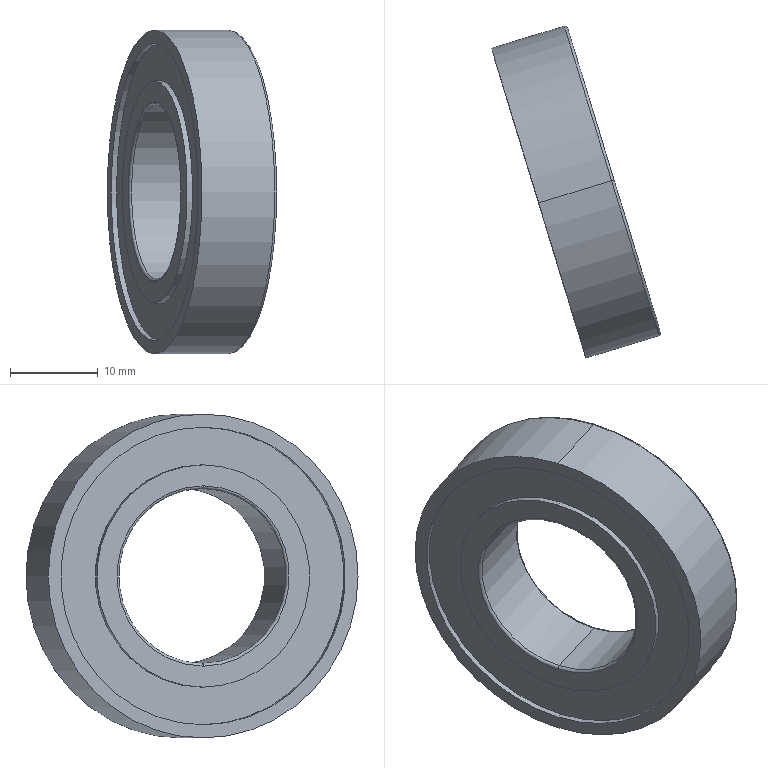Component | SolidWorks | v1ZHXTBGMWB6904ZZ_40SB1-1_v1ZHXTbearingB6904ZZSB1-1 | 1 solid | 24 faces | box 19.33 x 37.94 x 37 mm | volume 6323 mm3 | cylinder 12 | torus 6 | plane 6 | commonest cylinder face diameters 34 x4 25.4 x4 20 x2 37 x2
build123d program:
from build123d import *


with BuildPart() as part:
    # Sketch1 → Revolve1 (revolve)
    with BuildSketch(Plane.XY, mode=Mode.PRIVATE) as revolve1_sk:
        with BuildLine():
            Line((0, 18.5), (0, 17))
            Line((0, 17), (0.65, 17))
            Line((0.65, 17), (0.65, 12.7))
            Line((0.65, 12.7), (0, 12.7))
            Line((0, 12.7), (0, 10.3))
            ThreePointArc((0, 10.3), (0.08787, 10.088), (0.3, 10))
            Line((0.3, 10), (8.7, 10))
            ThreePointArc((8.7, 10), (8.912, 10.088), (9, 10.3))
            Line((9, 10.3), (9, 12.7))
            Line((9, 12.7), (8.35, 12.7))
            Line((8.35, 12.7), (8.35, 17))
            Line((8.35, 17), (9, 17))
            Line((9, 17), (9, 18.2))
            ThreePointArc((9, 18.2), (8.912, 18.412), (8.7, 18.5))
            Line((8.7, 18.5), (0, 18.5))
        make_face()
    revolve(revolve1_sk.sketch.rotate(Axis((9, 0, 0), (-1, 0, 0)), 270), axis=Axis((9, 0, 0), (-1, 0, 0)))


solid = part.part

# Placed as in the assembly
solid = solid.moved(Location((157.588, -238.137, 375.239), (15.285, 4.599, 16.35)))
STEP:
#1=CARTESIAN_POINT('',(6.543,-9.272,15.49));
#2=VERTEX_POINT('',#1);
#3=CARTESIAN_POINT('',(6.543,-9.272,14.057));
#4=VERTEX_POINT('',#3);
#5=CARTESIAN_POINT('',(6.543,-9.272,14.773));
#6=DIRECTION('',(-0.9565,-0.2918,-0.));
#7=DIRECTION('',(-0.,-0.,1.));
#8=AXIS2_PLACEMENT_3D('',#5,#6,#7);
#9=CIRCLE('',#8,0.7165);
#10=EDGE_CURVE('',#2,#4,#9,.T.);
#11=ORIENTED_EDGE('',*,*,#10,.T.);
#12=CARTESIAN_POINT('',(6.532,-9.276,14.045));
#13=VERTEX_POINT('',#12);
#14=CARTESIAN_POINT('',(6.532,-9.276,14.057));
#15=DIRECTION('',(-0.2918,0.9565,0.));
#16=DIRECTION('',(-0.9565,-0.2918,0.));
#17=AXIS2_PLACEMENT_3D('',#14,#15,#16);
#18=CIRCLE('',#17,0.01181);
#19=EDGE_CURVE('',#4,#13,#18,.T.);
#20=ORIENTED_EDGE('',*,*,#19,.T.);
#21=CARTESIAN_POINT('',(6.532,-9.276,15.502));
#22=VERTEX_POINT('',#21);
#23=CARTESIAN_POINT('',(6.532,-9.276,14.773));
#24=DIRECTION('',(-0.9565,-0.2918,-0.));
#25=DIRECTION('',(-0.,-0.,1.));
#26=AXIS2_PLACEMENT_3D('',#23,#24,#25);
#27=CIRCLE('',#26,0.7283);
#28=EDGE_CURVE('',#22,#13,#27,.T.);
#29=ORIENTED_EDGE('',*,*,#28,.F.);
#30=CARTESIAN_POINT('',(6.532,-9.276,15.49));
#31=DIRECTION('',(0.2918,-0.9565,-0.));
#32=DIRECTION('',(0.9565,0.2918,0.));
#33=AXIS2_PLACEMENT_3D('',#30,#31,#32);
#34=CIRCLE('',#33,0.01181);
#35=EDGE_CURVE('',#2,#22,#34,.T.);
#36=ORIENTED_EDGE('',*,*,#35,.F.);
#37=EDGE_LOOP('',(#11,#20,#29,#36));
#38=FACE_OUTER_BOUND('',#37,.T.);
#39=CARTESIAN_POINT('',(6.532,-9.276,14.773));
#40=DIRECTION('',(-0.9565,-0.2918,-0.));
#41=DIRECTION('',(-0.,-0.,1.));
#42=AXIS2_PLACEMENT_3D('',#39,#40,#41);
#43=TOROIDAL_SURFACE('',#42,0.7165,0.01181);
#44=ADVANCED_FACE('',(#38),#43,.T.);
#45=CARTESIAN_POINT('',(6.543,-9.272,14.104));
#46=VERTEX_POINT('',#45);
#47=CARTESIAN_POINT('',(6.543,-9.272,15.442));
#48=VERTEX_POINT('',#47);
#49=CARTESIAN_POINT('',(6.543,-9.272,14.773));
#50=DIRECTION('',(-0.9565,-0.2918,-0.));
#51=DIRECTION('',(-0.,-0.,1.));
#52=AXIS2_PLACEMENT_3D('',#49,#50,#51);
#53=CIRCLE('',#52,0.6693);
#54=EDGE_CURVE('',#46,#48,#53,.T.);
#55=ORIENTED_EDGE('',*,*,#54,.F.);
#56=CARTESIAN_POINT('',(6.519,-9.28,14.104));
#57=VERTEX_POINT('',#56);
#58=CARTESIAN_POINT('',(6.543,-9.272,14.104));
#59=DIRECTION('',(-0.9565,-0.2918,-0.));
#60=VECTOR('',#59,39.37);
#61=LINE('',#58,#60);
#62=EDGE_CURVE('',#46,#57,#61,.T.);
#63=ORIENTED_EDGE('',*,*,#62,.T.);
#64=CARTESIAN_POINT('',(6.519,-9.28,15.442));
#65=VERTEX_POINT('',#64);
#66=CARTESIAN_POINT('',(6.519,-9.28,14.773));
#67=DIRECTION('',(-0.9565,-0.2918,-0.));
#68=DIRECTION('',(-0.,-0.,1.));
#69=AXIS2_PLACEMENT_3D('',#66,#67,#68);
#70=CIRCLE('',#69,0.6693);
#71=EDGE_CURVE('',#57,#65,#70,.T.);
#72=ORIENTED_EDGE('',*,*,#71,.T.);
#73=CARTESIAN_POINT('',(6.543,-9.272,15.442));
#74=DIRECTION('',(-0.9565,-0.2918,-0.));
#75=VECTOR('',#74,39.37);
#76=LINE('',#73,#75);
#77=EDGE_CURVE('',#48,#65,#76,.T.);
#78=ORIENTED_EDGE('',*,*,#77,.F.);
#79=EDGE_LOOP('',(#55,#63,#72,#78));
#80=FACE_OUTER_BOUND('',#79,.T.);
#81=CARTESIAN_POINT('',(6.543,-9.272,14.773));
#82=DIRECTION('',(-0.9565,-0.2918,-0.));
#83=DIRECTION('',(-0.,-0.,1.));
#84=AXIS2_PLACEMENT_3D('',#81,#82,#83);
#85=CYLINDRICAL_SURFACE('',#84,0.6693);
#86=ADVANCED_FACE('',(#80),#85,.F.);
#87=CARTESIAN_POINT('',(6.543,-9.272,15.273));
#88=VERTEX_POINT('',#87);
#89=CARTESIAN_POINT('',(6.543,-9.272,14.273));
#90=VERTEX_POINT('',#89);
#91=CARTESIAN_POINT('',(6.543,-9.272,14.773));
#92=DIRECTION('',(-0.9565,-0.2918,-0.));
#93=DIRECTION('',(-0.,-0.,1.));
#94=AXIS2_PLACEMENT_3D('',#91,#92,#93);
#95=CIRCLE('',#94,0.5);
#96=EDGE_CURVE('',#88,#90,#95,.T.);
#97=ORIENTED_EDGE('',*,*,#96,.T.);
#98=CARTESIAN_POINT('',(6.519,-9.28,14.273));
#99=VERTEX_POINT('',#98);
#100=CARTESIAN_POINT('',(6.543,-9.272,14.273));
#101=DIRECTION('',(-0.9565,-0.2918,-0.));
#102=VECTOR('',#101,39.37);
#103=LINE('',#100,#102);
#104=EDGE_CURVE('',#90,#99,#103,.T.);
#105=ORIENTED_EDGE('',*,*,#104,.T.);
#106=CARTESIAN_POINT('',(6.519,-9.28,15.273));
#107=VERTEX_POINT('',#106);
#108=CARTESIAN_POINT('',(6.519,-9.28,14.773));
#109=DIRECTION('',(-0.9565,-0.2918,-0.));
#110=DIRECTION('',(-0.,-0.,1.));
#111=AXIS2_PLACEMENT_3D('',#108,#109,#110);
#112=CIRCLE('',#111,0.5);
#113=EDGE_CURVE('',#107,#99,#112,.T.);
#114=ORIENTED_EDGE('',*,*,#113,.F.);
#115=CARTESIAN_POINT('',(6.543,-9.272,15.273));
#116=DIRECTION('',(-0.9565,-0.2918,-0.));
#117=VECTOR('',#116,39.37);
#118=LINE('',#115,#117);
#119=EDGE_CURVE('',#88,#107,#118,.T.);
#120=ORIENTED_EDGE('',*,*,#119,.F.);
#121=EDGE_LOOP('',(#97,#105,#114,#120));
#122=FACE_OUTER_BOUND('',#121,.T.);
#123=CARTESIAN_POINT('',(6.543,-9.272,14.773));
#124=DIRECTION('',(-0.9565,-0.2918,-0.));
#125=DIRECTION('',(-0.,-0.,1.));
#126=AXIS2_PLACEMENT_3D('',#123,#124,#125);
#127=CYLINDRICAL_SURFACE('',#126,0.5);
#128=ADVANCED_FACE('',(#122),#127,.T.);
#129=CARTESIAN_POINT('',(6.532,-9.276,15.167));
#130=VERTEX_POINT('',#129);
#131=CARTESIAN_POINT('',(6.532,-9.276,14.379));
#132=VERTEX_POINT('',#131);
#133=CARTESIAN_POINT('',(6.532,-9.276,14.773));
#134=DIRECTION('',(-0.9565,-0.2918,-0.));
#135=DIRECTION('',(0.,-0.,1.));
#136=AXIS2_PLACEMENT_3D('',#133,#134,#135);
#137=CIRCLE('',#136,0.3937);
#138=EDGE_CURVE('',#130,#132,#137,.T.);
#139=ORIENTED_EDGE('',*,*,#138,.T.);
#140=CARTESIAN_POINT('',(6.543,-9.272,14.368));
#141=VERTEX_POINT('',#140);
#142=CARTESIAN_POINT('',(6.532,-9.276,14.368));
#143=DIRECTION('',(-0.2918,0.9565,0.));
#144=DIRECTION('',(-0.9565,-0.2918,0.));
#145=AXIS2_PLACEMENT_3D('',#142,#143,#144);
#146=CIRCLE('',#145,0.01181);
#147=EDGE_CURVE('',#132,#141,#146,.T.);
#148=ORIENTED_EDGE('',*,*,#147,.T.);
#149=CARTESIAN_POINT('',(6.543,-9.272,15.179));
#150=VERTEX_POINT('',#149);
#151=CARTESIAN_POINT('',(6.543,-9.272,14.773));
#152=DIRECTION('',(-0.9565,-0.2918,-0.));
#153=DIRECTION('',(-0.,-0.,1.));
#154=AXIS2_PLACEMENT_3D('',#151,#152,#153);
#155=CIRCLE('',#154,0.4055);
#156=EDGE_CURVE('',#150,#141,#155,.T.);
#157=ORIENTED_EDGE('',*,*,#156,.F.);
#158=CARTESIAN_POINT('',(6.532,-9.276,15.179));
#159=DIRECTION('',(0.2918,-0.9565,-0.));
#160=DIRECTION('',(0.9565,0.2918,0.));
#161=AXIS2_PLACEMENT_3D('',#158,#159,#160);
#162=CIRCLE('',#161,0.01181);
#163=EDGE_CURVE('',#130,#150,#162,.T.);
#164=ORIENTED_EDGE('',*,*,#163,.F.);
#165=EDGE_LOOP('',(#139,#148,#157,#164));
#166=FACE_OUTER_BOUND('',#165,.T.);
#167=CARTESIAN_POINT('',(6.532,-9.276,14.773));
#168=DIRECTION('',(-0.9565,-0.2918,-0.));
#169=DIRECTION('',(-0.,-0.,1.));
#170=AXIS2_PLACEMENT_3D('',#167,#168,#169);
#171=TOROIDAL_SURFACE('',#170,0.4055,0.01181);
#172=ADVANCED_FACE('',(#166),#171,.T.);
#173=CARTESIAN_POINT('',(6.532,-9.276,14.773));
#174=DIRECTION('',(-0.9565,-0.2918,-0.));
#175=DIRECTION('',(0.,-0.,1.));
#176=AXIS2_PLACEMENT_3D('',#173,#174,#175);
#177=CIRCLE('',#176,0.3937);
#178=EDGE_CURVE('',#132,#130,#177,.T.);
#179=ORIENTED_EDGE('',*,*,#178,.F.);
#180=CARTESIAN_POINT('',(6.216,-9.372,14.379));
#181=VERTEX_POINT('',#180);
#182=CARTESIAN_POINT('',(6.543,-9.272,14.379));
#183=DIRECTION('',(-0.9565,-0.2918,-0.));
#184=VECTOR('',#183,39.37);
#185=LINE('',#182,#184);
#186=EDGE_CURVE('',#132,#181,#185,.T.);
#187=ORIENTED_EDGE('',*,*,#186,.T.);
#188=CARTESIAN_POINT('',(6.216,-9.372,15.167));
#189=VERTEX_POINT('',#188);
#190=CARTESIAN_POINT('',(6.216,-9.372,14.773));
#191=DIRECTION('',(-0.9565,-0.2918,-0.));
#192=DIRECTION('',(0.,-0.,1.));
#193=AXIS2_PLACEMENT_3D('',#190,#191,#192);
#194=CIRCLE('',#193,0.3937);
#195=EDGE_CURVE('',#181,#189,#194,.T.);
#196=ORIENTED_EDGE('',*,*,#195,.T.);
#197=CARTESIAN_POINT('',(6.543,-9.272,15.167));
#198=DIRECTION('',(-0.9565,-0.2918,-0.));
#199=VECTOR('',#198,39.37);
#200=LINE('',#197,#199);
#201=EDGE_CURVE('',#130,#189,#200,.T.);
#202=ORIENTED_EDGE('',*,*,#201,.F.);
#203=EDGE_LOOP('',(#179,#187,#196,#202));
#204=FACE_OUTER_BOUND('',#203,.T.);
#205=CARTESIAN_POINT('',(6.543,-9.272,14.773));
#206=DIRECTION('',(-0.9565,-0.2918,-0.));
#207=DIRECTION('',(0.,-0.,1.));
#208=AXIS2_PLACEMENT_3D('',#205,#206,#207);
#209=CYLINDRICAL_SURFACE('',#208,0.3937);
#210=ADVANCED_FACE('',(#204),#209,.F.);
#211=CARTESIAN_POINT('',(6.204,-9.375,15.179));
#212=VERTEX_POINT('',#211);
#213=CARTESIAN_POINT('',(6.204,-9.375,14.368));
#214=VERTEX_POINT('',#213);
#215=CARTESIAN_POINT('',(6.204,-9.375,14.773));
#216=DIRECTION('',(-0.9565,-0.2918,-0.));
#217=DIRECTION('',(-0.,-0.,1.));
#218=AXIS2_PLACEMENT_3D('',#215,#216,#217);
#219=CIRCLE('',#218,0.4055);
#220=EDGE_CURVE('',#212,#214,#219,.T.);
#221=ORIENTED_EDGE('',*,*,#220,.T.);
#222=CARTESIAN_POINT('',(6.216,-9.372,14.368));
#223=DIRECTION('',(-0.2918,0.9565,0.));
#224=DIRECTION('',(-0.9565,-0.2918,0.));
#225=AXIS2_PLACEMENT_3D('',#222,#223,#224);
#226=CIRCLE('',#225,0.01181);
#227=EDGE_CURVE('',#214,#181,#226,.T.);
#228=ORIENTED_EDGE('',*,*,#227,.T.);
#229=CARTESIAN_POINT('',(6.216,-9.372,14.773));
#230=DIRECTION('',(-0.9565,-0.2918,-0.));
#231=DIRECTION('',(0.,-0.,1.));
#232=AXIS2_PLACEMENT_3D('',#229,#230,#231);
#233=CIRCLE('',#232,0.3937);
#234=EDGE_CURVE('',#189,#181,#233,.T.);
#235=ORIENTED_EDGE('',*,*,#234,.F.);
#236=CARTESIAN_POINT('',(6.216,-9.372,15.179));
#237=DIRECTION('',(0.2918,-0.9565,-0.));
#238=DIRECTION('',(0.9565,0.2918,0.));
#239=AXIS2_PLACEMENT_3D('',#236,#237,#238);
#240=CIRCLE('',#239,0.01181);
#241=EDGE_CURVE('',#212,#189,#240,.T.);
#242=ORIENTED_EDGE('',*,*,#241,.F.);
#243=EDGE_LOOP('',(#221,#228,#235,#242));
#244=FACE_OUTER_BOUND('',#243,.T.);
#245=CARTESIAN_POINT('',(6.216,-9.372,14.773));
#246=DIRECTION('',(-0.9565,-0.2918,-0.));
#247=DIRECTION('',(-0.,-0.,1.));
#248=AXIS2_PLACEMENT_3D('',#245,#246,#247);
#249=TOROIDAL_SURFACE('',#248,0.4055,0.01181);
#250=ADVANCED_FACE('',(#244),#249,.T.);
#251=CARTESIAN_POINT('',(6.229,-9.368,15.273));
#252=VERTEX_POINT('',#251);
#253=CARTESIAN_POINT('',(6.229,-9.368,14.273));
#254=VERTEX_POINT('',#253);
#255=CARTESIAN_POINT('',(6.229,-9.368,14.773));
#256=DIRECTION('',(-0.9565,-0.2918,-0.));
#257=DIRECTION('',(-0.,-0.,1.));
#258=AXIS2_PLACEMENT_3D('',#255,#256,#257);
#259=CIRCLE('',#258,0.5);
#260=EDGE_CURVE('',#252,#254,#259,.T.);
#261=ORIENTED_EDGE('',*,*,#260,.T.);
#262=CARTESIAN_POINT('',(6.204,-9.375,14.273));
#263=VERTEX_POINT('',#262);
#264=CARTESIAN_POINT('',(6.543,-9.272,14.273));
#265=DIRECTION('',(-0.9565,-0.2918,-0.));
#266=VECTOR('',#265,39.37);
#267=LINE('',#264,#266);
#268=EDGE_CURVE('',#254,#263,#267,.T.);
#269=ORIENTED_EDGE('',*,*,#268,.T.);
#270=CARTESIAN_POINT('',(6.204,-9.375,15.273));
#271=VERTEX_POINT('',#270);
#272=CARTESIAN_POINT('',(6.204,-9.375,14.773));
#273=DIRECTION('',(-0.9565,-0.2918,-0.));
#274=DIRECTION('',(-0.,-0.,1.));
#275=AXIS2_PLACEMENT_3D('',#272,#273,#274);
#276=CIRCLE('',#275,0.5);
#277=EDGE_CURVE('',#271,#263,#276,.T.);
#278=ORIENTED_EDGE('',*,*,#277,.F.);
#279=CARTESIAN_POINT('',(6.543,-9.272,15.273));
#280=DIRECTION('',(-0.9565,-0.2918,-0.));
#281=VECTOR('',#280,39.37);
#282=LINE('',#279,#281);
#283=EDGE_CURVE('',#252,#271,#282,.T.);
#284=ORIENTED_EDGE('',*,*,#283,.F.);
#285=EDGE_LOOP('',(#261,#269,#278,#284));
#286=FACE_OUTER_BOUND('',#285,.T.);
#287=CARTESIAN_POINT('',(6.543,-9.272,14.773));
#288=DIRECTION('',(-0.9565,-0.2918,-0.));
#289=DIRECTION('',(-0.,-0.,1.));
#290=AXIS2_PLACEMENT_3D('',#287,#288,#289);
#291=CYLINDRICAL_SURFACE('',#290,0.5);
#292=ADVANCED_FACE('',(#286),#291,.T.);
#293=CARTESIAN_POINT('',(6.229,-9.368,14.104));
#294=VERTEX_POINT('',#293);
#295=CARTESIAN_POINT('',(6.229,-9.368,15.442));
#296=VERTEX_POINT('',#295);
#297=CARTESIAN_POINT('',(6.229,-9.368,14.773));
#298=DIRECTION('',(-0.9565,-0.2918,-0.));
#299=DIRECTION('',(-0.,-0.,1.));
#300=AXIS2_PLACEMENT_3D('',#297,#298,#299);
#301=CIRCLE('',#300,0.6693);
#302=EDGE_CURVE('',#294,#296,#301,.T.);
#303=ORIENTED_EDGE('',*,*,#302,.F.);
#304=CARTESIAN_POINT('',(6.204,-9.375,14.104));
#305=VERTEX_POINT('',#304);
#306=CARTESIAN_POINT('',(6.543,-9.272,14.104));
#307=DIRECTION('',(-0.9565,-0.2918,-0.));
#308=VECTOR('',#307,39.37);
#309=LINE('',#306,#308);
#310=EDGE_CURVE('',#294,#305,#309,.T.);
#311=ORIENTED_EDGE('',*,*,#310,.T.);
#312=CARTESIAN_POINT('',(6.204,-9.375,15.442));
#313=VERTEX_POINT('',#312);
#314=CARTESIAN_POINT('',(6.204,-9.375,14.773));
#315=DIRECTION('',(-0.9565,-0.2918,-0.));
#316=DIRECTION('',(-0.,-0.,1.));
#317=AXIS2_PLACEMENT_3D('',#314,#315,#316);
#318=CIRCLE('',#317,0.6693);
#319=EDGE_CURVE('',#305,#313,#318,.T.);
#320=ORIENTED_EDGE('',*,*,#319,.T.);
#321=CARTESIAN_POINT('',(6.543,-9.272,15.442));
#322=DIRECTION('',(-0.9565,-0.2918,-0.));
#323=VECTOR('',#322,39.37);
#324=LINE('',#321,#323);
#325=EDGE_CURVE('',#296,#313,#324,.T.);
#326=ORIENTED_EDGE('',*,*,#325,.F.);
#327=EDGE_LOOP('',(#303,#311,#320,#326));
#328=FACE_OUTER_BOUND('',#327,.T.);
#329=CARTESIAN_POINT('',(6.543,-9.272,14.773));
#330=DIRECTION('',(-0.9565,-0.2918,-0.));
#331=DIRECTION('',(-0.,-0.,1.));
#332=AXIS2_PLACEMENT_3D('',#329,#330,#331);
#333=CYLINDRICAL_SURFACE('',#332,0.6693);
#334=ADVANCED_FACE('',(#328),#333,.F.);
#335=ORIENTED_EDGE('',*,*,#28,.T.);
#336=CARTESIAN_POINT('',(6.204,-9.375,14.045));
#337=VERTEX_POINT('',#336);
#338=CARTESIAN_POINT('',(6.543,-9.272,14.045));
#339=DIRECTION('',(-0.9565,-0.2918,-0.));
#340=VECTOR('',#339,39.37);
#341=LINE('',#338,#340);
#342=EDGE_CURVE('',#13,#337,#341,.T.);
#343=ORIENTED_EDGE('',*,*,#342,.T.);
#344=CARTESIAN_POINT('',(6.204,-9.375,15.502));
#345=VERTEX_POINT('',#344);
#346=CARTESIAN_POINT('',(6.204,-9.375,14.773));
#347=DIRECTION('',(-0.9565,-0.2918,-0.));
#348=DIRECTION('',(-0.,-0.,1.));
#349=AXIS2_PLACEMENT_3D('',#346,#347,#348);
#350=CIRCLE('',#349,0.7283);
#351=EDGE_CURVE('',#345,#337,#350,.T.);
#352=ORIENTED_EDGE('',*,*,#351,.F.);
#353=CARTESIAN_POINT('',(6.543,-9.272,15.502));
#354=DIRECTION('',(-0.9565,-0.2918,-0.));
#355=VECTOR('',#354,39.37);
#356=LINE('',#353,#355);
#357=EDGE_CURVE('',#22,#345,#356,.T.);
#358=ORIENTED_EDGE('',*,*,#357,.F.);
#359=EDGE_LOOP('',(#335,#343,#352,#358));
#360=FACE_OUTER_BOUND('',#359,.T.);
#361=CARTESIAN_POINT('',(6.543,-9.272,14.773));
#362=DIRECTION('',(-0.9565,-0.2918,-0.));
#363=DIRECTION('',(-0.,-0.,1.));
#364=AXIS2_PLACEMENT_3D('',#361,#362,#363);
#365=CYLINDRICAL_SURFACE('',#364,0.7283);
#366=ADVANCED_FACE('',(#360),#365,.T.);
#367=ORIENTED_EDGE('',*,*,#342,.F.);
#368=CARTESIAN_POINT('',(6.532,-9.276,14.773));
#369=DIRECTION('',(-0.9565,-0.2918,-0.));
#370=DIRECTION('',(-0.,-0.,1.));
#371=AXIS2_PLACEMENT_3D('',#368,#369,#370);
#372=CIRCLE('',#371,0.7283);
#373=EDGE_CURVE('',#13,#22,#372,.T.);
#374=ORIENTED_EDGE('',*,*,#373,.T.);
#375=ORIENTED_EDGE('',*,*,#357,.T.);
#376=CARTESIAN_POINT('',(6.204,-9.375,14.773));
#377=DIRECTION('',(-0.9565,-0.2918,-0.));
#378=DIRECTION('',(-0.,-0.,1.));
#379=AXIS2_PLACEMENT_3D('',#376,#377,#378);
#380=CIRCLE('',#379,0.7283);
#381=EDGE_CURVE('',#337,#345,#380,.T.);
#382=ORIENTED_EDGE('',*,*,#381,.F.);
#383=EDGE_LOOP('',(#367,#374,#375,#382));
#384=FACE_OUTER_BOUND('',#383,.T.);
#385=CARTESIAN_POINT('',(6.543,-9.272,14.773));
#386=DIRECTION('',(-0.9565,-0.2918,-0.));
#387=DIRECTION('',(-0.,-0.,1.));
#388=AXIS2_PLACEMENT_3D('',#385,#386,#387);
#389=CYLINDRICAL_SURFACE('',#388,0.7283);
#390=ADVANCED_FACE('',(#384),#389,.T.);
#391=CARTESIAN_POINT('',(6.204,-9.375,14.773));
#392=DIRECTION('',(-0.9565,-0.2918,-0.));
#393=DIRECTION('',(-0.,-0.,1.));
#394=AXIS2_PLACEMENT_3D('',#391,#392,#393);
#395=CIRCLE('',#394,0.6693);
#396=EDGE_CURVE('',#313,#305,#395,.T.);
#397=ORIENTED_EDGE('',*,*,#396,.F.);
#398=ORIENTED_EDGE('',*,*,#319,.F.);
#399=EDGE_LOOP('',(#397,#398));
#400=FACE_BOUND('',#399,.T.);
#401=ORIENTED_EDGE('',*,*,#351,.T.);
#402=ORIENTED_EDGE('',*,*,#381,.T.);
#403=EDGE_LOOP('',(#401,#402));
#404=FACE_OUTER_BOUND('',#403,.T.);
#405=CARTESIAN_POINT('',(5.992,-8.679,14.773));
#406=DIRECTION('',(0.9565,0.2918,0.));
#407=DIRECTION('',(0.,0.,-1.));
#408=AXIS2_PLACEMENT_3D('',#405,#406,#407);
#409=PLANE('',#408);
#410=ADVANCED_FACE('',(#400,#404),#409,.F.);
#411=ORIENTED_EDGE('',*,*,#310,.F.);
#412=CARTESIAN_POINT('',(6.229,-9.368,14.773));
#413=DIRECTION('',(-0.9565,-0.2918,-0.));
#414=DIRECTION('',(-0.,-0.,1.));
#415=AXIS2_PLACEMENT_3D('',#412,#413,#414);
#416=CIRCLE('',#415,0.6693);
#417=EDGE_CURVE('',#296,#294,#416,.T.);
#418=ORIENTED_EDGE('',*,*,#417,.F.);
#419=ORIENTED_EDGE('',*,*,#325,.T.);
#420=ORIENTED_EDGE('',*,*,#396,.T.);
#421=EDGE_LOOP('',(#411,#418,#419,#420));
#422=FACE_OUTER_BOUND('',#421,.T.);
#423=CARTESIAN_POINT('',(6.543,-9.272,14.773));
#424=DIRECTION('',(-0.9565,-0.2918,-0.));
#425=DIRECTION('',(-0.,-0.,1.));
#426=AXIS2_PLACEMENT_3D('',#423,#424,#425);
#427=CYLINDRICAL_SURFACE('',#426,0.6693);
#428=ADVANCED_FACE('',(#422),#427,.F.);
#429=ORIENTED_EDGE('',*,*,#260,.F.);
#430=CARTESIAN_POINT('',(6.229,-9.368,14.773));
#431=DIRECTION('',(-0.9565,-0.2918,-0.));
#432=DIRECTION('',(-0.,-0.,1.));
#433=AXIS2_PLACEMENT_3D('',#430,#431,#432);
#434=CIRCLE('',#433,0.5);
#435=EDGE_CURVE('',#254,#252,#434,.T.);
#436=ORIENTED_EDGE('',*,*,#435,.F.);
#437=EDGE_LOOP('',(#429,#436));
#438=FACE_BOUND('',#437,.T.);
#439=ORIENTED_EDGE('',*,*,#417,.T.);
#440=ORIENTED_EDGE('',*,*,#302,.T.);
#441=EDGE_LOOP('',(#439,#440));
#442=FACE_OUTER_BOUND('',#441,.T.);
#443=CARTESIAN_POINT('',(6.033,-8.728,14.773));
#444=DIRECTION('',(0.9565,0.2918,0.));
#445=DIRECTION('',(0.,0.,-1.));
#446=AXIS2_PLACEMENT_3D('',#443,#444,#445);
#447=PLANE('',#446);
#448=ADVANCED_FACE('',(#438,#442),#447,.F.);
#449=ORIENTED_EDGE('',*,*,#268,.F.);
#450=ORIENTED_EDGE('',*,*,#435,.T.);
#451=ORIENTED_EDGE('',*,*,#283,.T.);
#452=CARTESIAN_POINT('',(6.204,-9.375,14.773));
#453=DIRECTION('',(-0.9565,-0.2918,-0.));
#454=DIRECTION('',(-0.,-0.,1.));
#455=AXIS2_PLACEMENT_3D('',#452,#453,#454);
#456=CIRCLE('',#455,0.5);
#457=EDGE_CURVE('',#263,#271,#456,.T.);
#458=ORIENTED_EDGE('',*,*,#457,.F.);
#459=EDGE_LOOP('',(#449,#450,#451,#458));
#460=FACE_OUTER_BOUND('',#459,.T.);
#461=CARTESIAN_POINT('',(6.543,-9.272,14.773));
#462=DIRECTION('',(-0.9565,-0.2918,-0.));
#463=DIRECTION('',(-0.,-0.,1.));
#464=AXIS2_PLACEMENT_3D('',#461,#462,#463);
#465=CYLINDRICAL_SURFACE('',#464,0.5);
#466=ADVANCED_FACE('',(#460),#465,.T.);
#467=ORIENTED_EDGE('',*,*,#220,.F.);
#468=CARTESIAN_POINT('',(6.204,-9.375,14.773));
#469=DIRECTION('',(-0.9565,-0.2918,-0.));
#470=DIRECTION('',(-0.,-0.,1.));
#471=AXIS2_PLACEMENT_3D('',#468,#469,#470);
#472=CIRCLE('',#471,0.4055);
#473=EDGE_CURVE('',#214,#212,#472,.T.);
#474=ORIENTED_EDGE('',*,*,#473,.F.);
#475=EDGE_LOOP('',(#467,#474));
#476=FACE_BOUND('',#475,.T.);
#477=ORIENTED_EDGE('',*,*,#277,.T.);
#478=ORIENTED_EDGE('',*,*,#457,.T.);
#479=EDGE_LOOP('',(#477,#478));
#480=FACE_OUTER_BOUND('',#479,.T.);
#481=CARTESIAN_POINT('',(6.058,-8.897,14.773));
#482=DIRECTION('',(0.9565,0.2918,0.));
#483=DIRECTION('',(0.,0.,-1.));
#484=AXIS2_PLACEMENT_3D('',#481,#482,#483);
#485=PLANE('',#484);
#486=ADVANCED_FACE('',(#476,#480),#485,.F.);
#487=ORIENTED_EDGE('',*,*,#227,.F.);
#488=ORIENTED_EDGE('',*,*,#473,.T.);
#489=ORIENTED_EDGE('',*,*,#241,.T.);
#490=ORIENTED_EDGE('',*,*,#195,.F.);
#491=EDGE_LOOP('',(#487,#488,#489,#490));
#492=FACE_OUTER_BOUND('',#491,.T.);
#493=CARTESIAN_POINT('',(6.216,-9.372,14.773));
#494=DIRECTION('',(-0.9565,-0.2918,-0.));
#495=DIRECTION('',(-0.,-0.,1.));
#496=AXIS2_PLACEMENT_3D('',#493,#494,#495);
#497=TOROIDAL_SURFACE('',#496,0.4055,0.01181);
#498=ADVANCED_FACE('',(#492),#497,.T.);
#499=ORIENTED_EDGE('',*,*,#186,.F.);
#500=ORIENTED_EDGE('',*,*,#138,.F.);
#501=ORIENTED_EDGE('',*,*,#201,.T.);
#502=ORIENTED_EDGE('',*,*,#234,.T.);
#503=EDGE_LOOP('',(#499,#500,#501,#502));
#504=FACE_OUTER_BOUND('',#503,.T.);
#505=CARTESIAN_POINT('',(6.543,-9.272,14.773));
#506=DIRECTION('',(-0.9565,-0.2918,-0.));
#507=DIRECTION('',(0.,-0.,1.));
#508=AXIS2_PLACEMENT_3D('',#505,#506,#507);
#509=CYLINDRICAL_SURFACE('',#508,0.3937);
#510=ADVANCED_FACE('',(#504),#509,.F.);
#511=ORIENTED_EDGE('',*,*,#147,.F.);
#512=ORIENTED_EDGE('',*,*,#178,.T.);
#513=ORIENTED_EDGE('',*,*,#163,.T.);
#514=CARTESIAN_POINT('',(6.543,-9.272,14.773));
#515=DIRECTION('',(-0.9565,-0.2918,-0.));
#516=DIRECTION('',(-0.,-0.,1.));
#517=AXIS2_PLACEMENT_3D('',#514,#515,#516);
#518=CIRCLE('',#517,0.4055);
#519=EDGE_CURVE('',#141,#150,#518,.T.);
#520=ORIENTED_EDGE('',*,*,#519,.F.);
#521=EDGE_LOOP('',(#511,#512,#513,#520));
#522=FACE_OUTER_BOUND('',#521,.T.);
#523=CARTESIAN_POINT('',(6.532,-9.276,14.773));
#524=DIRECTION('',(-0.9565,-0.2918,-0.));
#525=DIRECTION('',(-0.,-0.,1.));
#526=AXIS2_PLACEMENT_3D('',#523,#524,#525);
#527=TOROIDAL_SURFACE('',#526,0.4055,0.01181);
#528=ADVANCED_FACE('',(#522),#527,.T.);
#529=ORIENTED_EDGE('',*,*,#96,.F.);
#530=CARTESIAN_POINT('',(6.543,-9.272,14.773));
#531=DIRECTION('',(-0.9565,-0.2918,-0.));
#532=DIRECTION('',(-0.,-0.,1.));
#533=AXIS2_PLACEMENT_3D('',#530,#531,#532);
#534=CIRCLE('',#533,0.5);
#535=EDGE_CURVE('',#90,#88,#534,.T.);
#536=ORIENTED_EDGE('',*,*,#535,.F.);
#537=EDGE_LOOP('',(#529,#536));
#538=FACE_OUTER_BOUND('',#537,.T.);
#539=ORIENTED_EDGE('',*,*,#156,.T.);
#540=ORIENTED_EDGE('',*,*,#519,.T.);
#541=EDGE_LOOP('',(#539,#540));
#542=FACE_BOUND('',#541,.T.);
#543=CARTESIAN_POINT('',(6.425,-8.884,14.773));
#544=DIRECTION('',(-0.9565,-0.2918,-0.));
#545=DIRECTION('',(-0.,-0.,1.));
#546=AXIS2_PLACEMENT_3D('',#543,#544,#545);
#547=PLANE('',#546);
#548=ADVANCED_FACE('',(#538,#542),#547,.F.);
#549=ORIENTED_EDGE('',*,*,#104,.F.);
#550=ORIENTED_EDGE('',*,*,#535,.T.);
#551=ORIENTED_EDGE('',*,*,#119,.T.);
#552=CARTESIAN_POINT('',(6.519,-9.28,14.773));
#553=DIRECTION('',(-0.9565,-0.2918,-0.));
#554=DIRECTION('',(-0.,-0.,1.));
#555=AXIS2_PLACEMENT_3D('',#552,#553,#554);
#556=CIRCLE('',#555,0.5);
#557=EDGE_CURVE('',#99,#107,#556,.T.);
#558=ORIENTED_EDGE('',*,*,#557,.F.);
#559=EDGE_LOOP('',(#549,#550,#551,#558));
#560=FACE_OUTER_BOUND('',#559,.T.);
#561=CARTESIAN_POINT('',(6.543,-9.272,14.773));
#562=DIRECTION('',(-0.9565,-0.2918,-0.));
#563=DIRECTION('',(-0.,-0.,1.));
#564=AXIS2_PLACEMENT_3D('',#561,#562,#563);
#565=CYLINDRICAL_SURFACE('',#564,0.5);
#566=ADVANCED_FACE('',(#560),#565,.T.);
#567=CARTESIAN_POINT('',(6.519,-9.28,14.773));
#568=DIRECTION('',(-0.9565,-0.2918,-0.));
#569=DIRECTION('',(-0.,-0.,1.));
#570=AXIS2_PLACEMENT_3D('',#567,#568,#569);
#571=CIRCLE('',#570,0.6693);
#572=EDGE_CURVE('',#65,#57,#571,.T.);
#573=ORIENTED_EDGE('',*,*,#572,.F.);
#574=ORIENTED_EDGE('',*,*,#71,.F.);
#575=EDGE_LOOP('',(#573,#574));
#576=FACE_OUTER_BOUND('',#575,.T.);
#577=ORIENTED_EDGE('',*,*,#113,.T.);
#578=ORIENTED_EDGE('',*,*,#557,.T.);
#579=EDGE_LOOP('',(#577,#578));
#580=FACE_BOUND('',#579,.T.);
#581=CARTESIAN_POINT('',(6.373,-8.801,14.773));
#582=DIRECTION('',(-0.9565,-0.2918,-0.));
#583=DIRECTION('',(-0.,-0.,1.));
#584=AXIS2_PLACEMENT_3D('',#581,#582,#583);
#585=PLANE('',#584);
#586=ADVANCED_FACE('',(#576,#580),#585,.F.);
#587=ORIENTED_EDGE('',*,*,#62,.F.);
#588=CARTESIAN_POINT('',(6.543,-9.272,14.773));
#589=DIRECTION('',(-0.9565,-0.2918,-0.));
#590=DIRECTION('',(-0.,-0.,1.));
#591=AXIS2_PLACEMENT_3D('',#588,#589,#590);
#592=CIRCLE('',#591,0.6693);
#593=EDGE_CURVE('',#48,#46,#592,.T.);
#594=ORIENTED_EDGE('',*,*,#593,.F.);
#595=ORIENTED_EDGE('',*,*,#77,.T.);
#596=ORIENTED_EDGE('',*,*,#572,.T.);
#597=EDGE_LOOP('',(#587,#594,#595,#596));
#598=FACE_OUTER_BOUND('',#597,.T.);
#599=CARTESIAN_POINT('',(6.543,-9.272,14.773));
#600=DIRECTION('',(-0.9565,-0.2918,-0.));
#601=DIRECTION('',(-0.,-0.,1.));
#602=AXIS2_PLACEMENT_3D('',#599,#600,#601);
#603=CYLINDRICAL_SURFACE('',#602,0.6693);
#604=ADVANCED_FACE('',(#598),#603,.F.);
#605=ORIENTED_EDGE('',*,*,#10,.F.);
#606=CARTESIAN_POINT('',(6.543,-9.272,14.773));
#607=DIRECTION('',(-0.9565,-0.2918,-0.));
#608=DIRECTION('',(-0.,-0.,1.));
#609=AXIS2_PLACEMENT_3D('',#606,#607,#608);
#610=CIRCLE('',#609,0.7165);
#611=EDGE_CURVE('',#4,#2,#610,.T.);
#612=ORIENTED_EDGE('',*,*,#611,.F.);
#613=EDGE_LOOP('',(#605,#612));
#614=FACE_OUTER_BOUND('',#613,.T.);
#615=ORIENTED_EDGE('',*,*,#593,.T.);
#616=ORIENTED_EDGE('',*,*,#54,.T.);
#617=EDGE_LOOP('',(#615,#616));
#618=FACE_BOUND('',#617,.T.);
#619=CARTESIAN_POINT('',(6.348,-8.632,14.773));
#620=DIRECTION('',(-0.9565,-0.2918,-0.));
#621=DIRECTION('',(-0.,-0.,1.));
#622=AXIS2_PLACEMENT_3D('',#619,#620,#621);
#623=PLANE('',#622);
#624=ADVANCED_FACE('',(#614,#618),#623,.F.);
#625=ORIENTED_EDGE('',*,*,#19,.F.);
#626=ORIENTED_EDGE('',*,*,#611,.T.);
#627=ORIENTED_EDGE('',*,*,#35,.T.);
#628=ORIENTED_EDGE('',*,*,#373,.F.);
#629=EDGE_LOOP('',(#625,#626,#627,#628));
#630=FACE_OUTER_BOUND('',#629,.T.);
#631=CARTESIAN_POINT('',(6.532,-9.276,14.773));
#632=DIRECTION('',(-0.9565,-0.2918,-0.));
#633=DIRECTION('',(-0.,-0.,1.));
#634=AXIS2_PLACEMENT_3D('',#631,#632,#633);
#635=TOROIDAL_SURFACE('',#634,0.7165,0.01181);
#636=ADVANCED_FACE('',(#630),#635,.T.);
#637=CLOSED_SHELL('',(#44,#86,#128,#172,#210,#250,#292,#334,#366,#390,#410,#428,#448,#466,#486,#498,#510,#528,#548,#566,#586,#604,#624,#636));
#638=MANIFOLD_SOLID_BREP('',#637);
#639=CARTESIAN_POINT('',(0.,0.,0.));
#640=DIRECTION('',(0.,0.,1.));
#641=DIRECTION('',(1.,0.,0.));
#642=AXIS2_PLACEMENT_3D('',#639,#640,#641);
#643=(LENGTH_UNIT()NAMED_UNIT(*)SI_UNIT($,.METRE.));
#644=LENGTH_MEASURE_WITH_UNIT(LENGTH_MEASURE(0.0254),#643);
#645=DIMENSIONAL_EXPONENTS(1.,0.,0.,0.,0.,0.,0.);
#646=(CONVERSION_BASED_UNIT('',#644)LENGTH_UNIT()NAMED_UNIT(#645));
#647=UNCERTAINTY_MEASURE_WITH_UNIT(LENGTH_MEASURE(0.00001),#646,'','');
#648=(NAMED_UNIT(*)PLANE_ANGLE_UNIT()SI_UNIT($,.RADIAN.));
#649=(NAMED_UNIT(*)SI_UNIT($,.STERADIAN.)SOLID_ANGLE_UNIT());
#650=(GEOMETRIC_REPRESENTATION_CONTEXT(3)GLOBAL_UNCERTAINTY_ASSIGNED_CONTEXT((#647))GLOBAL_UNIT_ASSIGNED_CONTEXT((#646,#648,#649))REPRESENTATION_CONTEXT('',''));
#651=ADVANCED_BREP_SHAPE_REPRESENTATION('',(#638,#642),#650);
#652=COLOUR_RGB('',0.7922,0.8196,0.9333);
#653=FILL_AREA_STYLE_COLOUR('',#652);
#654=FILL_AREA_STYLE('',(#653));
#655=SURFACE_STYLE_FILL_AREA(#654);
#656=SURFACE_SIDE_STYLE('',(#655));
#657=SURFACE_STYLE_USAGE(.BOTH.,#656);
#658=PRESENTATION_STYLE_ASSIGNMENT((#657));
#659=STYLED_ITEM('',(#658),#638);
#660=(LENGTH_UNIT()NAMED_UNIT(*)SI_UNIT($,.METRE.));
#661=LENGTH_MEASURE_WITH_UNIT(LENGTH_MEASURE(0.0254),#660);
#662=DIMENSIONAL_EXPONENTS(1.,0.,0.,0.,0.,0.,0.);
#663=(CONVERSION_BASED_UNIT('',#661)LENGTH_UNIT()NAMED_UNIT(#662));
#664=UNCERTAINTY_MEASURE_WITH_UNIT(LENGTH_MEASURE(0.00001),#663,'','');
#665=(NAMED_UNIT(*)PLANE_ANGLE_UNIT()SI_UNIT($,.RADIAN.));
#666=(NAMED_UNIT(*)SI_UNIT($,.STERADIAN.)SOLID_ANGLE_UNIT());
#667=(GEOMETRIC_REPRESENTATION_CONTEXT(3)GLOBAL_UNCERTAINTY_ASSIGNED_CONTEXT((#664))GLOBAL_UNIT_ASSIGNED_CONTEXT((#663,#665,#666))REPRESENTATION_CONTEXT('',''));
#668=MECHANICAL_DESIGN_GEOMETRIC_PRESENTATION_REPRESENTATION('',(#659),#667);
#669=PRESENTATION_LAYER_ASSIGNMENT('','',(#659));